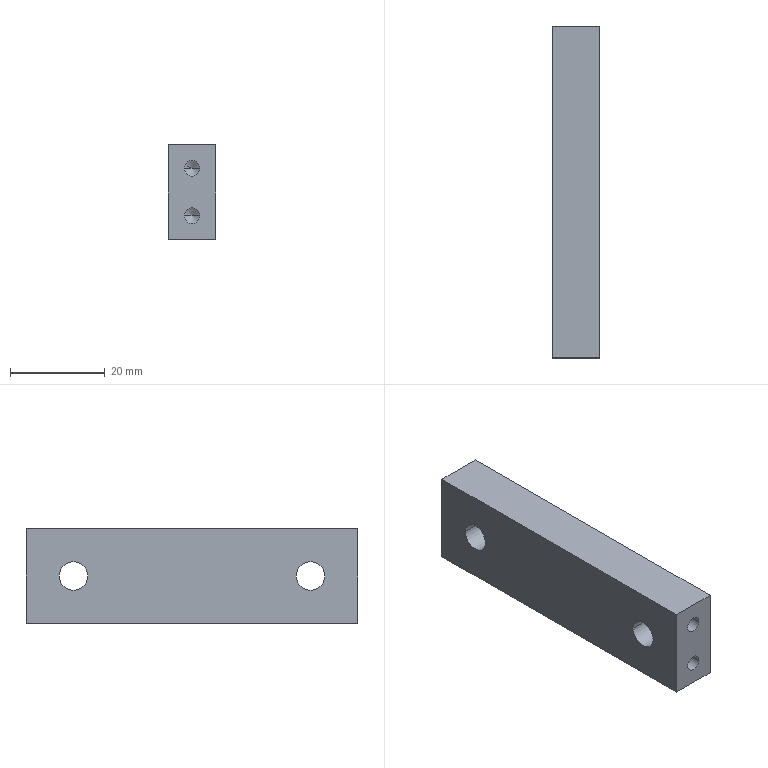Component | SolidWorks | EpoxyBoardSupportBlock-1 | 1 solid | 26 faces | box 10 x 70 x 20 mm | volume 13010 mm3 | cylinder 12 | cone 8 | plane 6 | commonest cylinder face diameters 3.3 x8 6 x4
build123d program:
from build123d import *

# Parameters (mm, degrees)
SKETCH1_W             = 70
SKETCH1_H             = 20
BOSS_EXTRUDE1_DEPTH   = 5
M6_TAPPED_HOLE1_D     = 6
M4_TAPPED_HOLE1_D     = 3.3
M4_TAPPED_HOLE1_DEPTH = 12.1
M4_TAPPED_HOLE1_TIP   = 0.9526
M4_TAPPED_HOLE2_D     = 3.3
M4_TAPPED_HOLE2_DEPTH = 12.1
M4_TAPPED_HOLE2_TIP   = 0.9526


with BuildPart() as part:
    # Sketch1 → Boss-Extrude1 (new, symmetric)
    with BuildSketch(Plane.XY):
        with Locations((35, 10)):
            Rectangle(SKETCH1_W, SKETCH1_H)
    extrude(amount=BOSS_EXTRUDE1_DEPTH, both=True)

    # M6 Tapped Hole1 (through all)
    with Locations(Plane(origin=(10, 10, 5), x_dir=(1, 0, 0), z_dir=(0, 0, 1))):
        with Locations((0, 0), (50, 0)):
            Hole(M6_TAPPED_HOLE1_D / 2)

    # M4 Tapped Hole1
    with Locations(Plane(origin=(0, 15, 0), x_dir=(0, 0, -1), z_dir=(-1, 0, 0))):
        with Locations((0, 0), (0, 10)):
            Hole(M4_TAPPED_HOLE1_D / 2, depth=M4_TAPPED_HOLE1_DEPTH)
            with Locations((0, 0, -(M4_TAPPED_HOLE1_DEPTH + M4_TAPPED_HOLE1_TIP / 2))):  # 120° drill point
                Cone(0, M4_TAPPED_HOLE1_D / 2, M4_TAPPED_HOLE1_TIP, mode=Mode.SUBTRACT)

    # M4 Tapped Hole2
    with Locations(Plane(origin=(70, 15, 0), x_dir=(0, 0, 1), z_dir=(1, 0, 0))):
        with Locations((0, 0), (0, 10)):
            Hole(M4_TAPPED_HOLE2_D / 2, depth=M4_TAPPED_HOLE2_DEPTH)
            with Locations((0, 0, -(M4_TAPPED_HOLE2_DEPTH + M4_TAPPED_HOLE2_TIP / 2))):  # 120° drill point
                Cone(0, M4_TAPPED_HOLE2_D / 2, M4_TAPPED_HOLE2_TIP, mode=Mode.SUBTRACT)


solid = part.part

# Placed as in the assembly
solid = solid.moved(Location((-28.341, 72.185, -51.775), (90, -90, 0)))
STEP:
#1=COLOUR_RGB('',0.7922,0.8196,0.9333);
#2=FILL_AREA_STYLE_COLOUR('',#1);
#3=FILL_AREA_STYLE('',(#2));
#4=SURFACE_STYLE_FILL_AREA(#3);
#5=SURFACE_SIDE_STYLE('',(#4));
#6=SURFACE_STYLE_USAGE(.BOTH.,#5);
#7=PRESENTATION_STYLE_ASSIGNMENT((#6));
#8=CARTESIAN_POINT('',(-1.051,0.5624,-1.842));
#9=VERTEX_POINT('',#8);
#10=CARTESIAN_POINT('',(-1.181,0.5624,-1.842));
#11=VERTEX_POINT('',#10);
#12=CARTESIAN_POINT('',(-1.116,0.5624,-1.842));
#13=DIRECTION('',(0.,-1.,0.));
#14=DIRECTION('',(-1.,0.,0.));
#15=AXIS2_PLACEMENT_3D('',#12,#13,#14);
#16=CIRCLE('',#15,0.06496);
#17=EDGE_CURVE('',#9,#11,#16,.T.);
#18=ORIENTED_EDGE('',*,*,#17,.F.);
#19=CARTESIAN_POINT('',(-1.051,0.08603,-1.842));
#20=VERTEX_POINT('',#19);
#21=CARTESIAN_POINT('',(-1.051,0.08603,-1.842));
#22=DIRECTION('',(0.,-1.,0.));
#23=VECTOR('',#22,39.37);
#24=LINE('',#21,#23);
#25=EDGE_CURVE('',#9,#20,#24,.T.);
#26=ORIENTED_EDGE('',*,*,#25,.T.);
#27=CARTESIAN_POINT('',(-1.181,0.08603,-1.842));
#28=VERTEX_POINT('',#27);
#29=CARTESIAN_POINT('',(-1.116,0.08603,-1.842));
#30=DIRECTION('',(0.,-1.,0.));
#31=DIRECTION('',(-1.,0.,0.));
#32=AXIS2_PLACEMENT_3D('',#29,#30,#31);
#33=CIRCLE('',#32,0.06496);
#34=EDGE_CURVE('',#20,#28,#33,.T.);
#35=ORIENTED_EDGE('',*,*,#34,.T.);
#36=CARTESIAN_POINT('',(-1.181,0.08603,-1.842));
#37=DIRECTION('',(0.,-1.,0.));
#38=VECTOR('',#37,39.37);
#39=LINE('',#36,#38);
#40=EDGE_CURVE('',#11,#28,#39,.T.);
#41=ORIENTED_EDGE('',*,*,#40,.F.);
#42=EDGE_LOOP('',(#18,#26,#35,#41));
#43=FACE_OUTER_BOUND('',#42,.T.);
#44=CARTESIAN_POINT('',(-1.116,0.08603,-1.842));
#45=DIRECTION('',(0.,-1.,0.));
#46=DIRECTION('',(-1.,0.,0.));
#47=AXIS2_PLACEMENT_3D('',#44,#45,#46);
#48=CYLINDRICAL_SURFACE('',#47,0.06496);
#49=ADVANCED_FACE('',(#43),#48,.F.);
#50=CARTESIAN_POINT('',(-1.116,0.5999,-1.842));
#51=VERTEX_POINT('',#50);
#52=CARTESIAN_POINT('',(-1.181,0.5624,-1.842));
#53=DIRECTION('',(-0.866,-0.5,0.));
#54=VECTOR('',#53,39.37);
#55=LINE('',#52,#54);
#56=EDGE_CURVE('',#51,#11,#55,.T.);
#57=ORIENTED_EDGE('',*,*,#56,.F.);
#58=CARTESIAN_POINT('',(-1.051,0.5624,-1.842));
#59=DIRECTION('',(0.866,-0.5,0.));
#60=VECTOR('',#59,39.37);
#61=LINE('',#58,#60);
#62=EDGE_CURVE('',#51,#9,#61,.T.);
#63=ORIENTED_EDGE('',*,*,#62,.T.);
#64=ORIENTED_EDGE('',*,*,#17,.T.);
#65=EDGE_LOOP('',(#57,#63,#64));
#66=FACE_OUTER_BOUND('',#65,.T.);
#67=CARTESIAN_POINT('',(-1.116,0.5624,-1.842));
#68=DIRECTION('',(0.,-1.,0.));
#69=DIRECTION('',(-1.,0.,0.));
#70=AXIS2_PLACEMENT_3D('',#67,#68,#69);
#71=CONICAL_SURFACE('',#70,0.06496,1.047);
#72=ADVANCED_FACE('',(#66),#71,.F.);
#73=CARTESIAN_POINT('',(-1.051,0.5624,-1.448));
#74=VERTEX_POINT('',#73);
#75=CARTESIAN_POINT('',(-1.181,0.5624,-1.448));
#76=VERTEX_POINT('',#75);
#77=CARTESIAN_POINT('',(-1.116,0.5624,-1.448));
#78=DIRECTION('',(0.,-1.,0.));
#79=DIRECTION('',(-1.,0.,0.));
#80=AXIS2_PLACEMENT_3D('',#77,#78,#79);
#81=CIRCLE('',#80,0.06496);
#82=EDGE_CURVE('',#74,#76,#81,.T.);
#83=ORIENTED_EDGE('',*,*,#82,.F.);
#84=CARTESIAN_POINT('',(-1.051,0.08603,-1.448));
#85=VERTEX_POINT('',#84);
#86=CARTESIAN_POINT('',(-1.051,0.08603,-1.448));
#87=DIRECTION('',(0.,-1.,0.));
#88=VECTOR('',#87,39.37);
#89=LINE('',#86,#88);
#90=EDGE_CURVE('',#74,#85,#89,.T.);
#91=ORIENTED_EDGE('',*,*,#90,.T.);
#92=CARTESIAN_POINT('',(-1.181,0.08603,-1.448));
#93=VERTEX_POINT('',#92);
#94=CARTESIAN_POINT('',(-1.116,0.08603,-1.448));
#95=DIRECTION('',(0.,-1.,0.));
#96=DIRECTION('',(-1.,0.,0.));
#97=AXIS2_PLACEMENT_3D('',#94,#95,#96);
#98=CIRCLE('',#97,0.06496);
#99=EDGE_CURVE('',#85,#93,#98,.T.);
#100=ORIENTED_EDGE('',*,*,#99,.T.);
#101=CARTESIAN_POINT('',(-1.181,0.08603,-1.448));
#102=DIRECTION('',(0.,-1.,0.));
#103=VECTOR('',#102,39.37);
#104=LINE('',#101,#103);
#105=EDGE_CURVE('',#76,#93,#104,.T.);
#106=ORIENTED_EDGE('',*,*,#105,.F.);
#107=EDGE_LOOP('',(#83,#91,#100,#106));
#108=FACE_OUTER_BOUND('',#107,.T.);
#109=CARTESIAN_POINT('',(-1.116,0.08603,-1.448));
#110=DIRECTION('',(0.,-1.,0.));
#111=DIRECTION('',(-1.,0.,0.));
#112=AXIS2_PLACEMENT_3D('',#109,#110,#111);
#113=CYLINDRICAL_SURFACE('',#112,0.06496);
#114=ADVANCED_FACE('',(#108),#113,.F.);
#115=CARTESIAN_POINT('',(-1.116,0.5999,-1.448));
#116=VERTEX_POINT('',#115);
#117=CARTESIAN_POINT('',(-1.181,0.5624,-1.448));
#118=DIRECTION('',(-0.866,-0.5,0.));
#119=VECTOR('',#118,39.37);
#120=LINE('',#117,#119);
#121=EDGE_CURVE('',#116,#76,#120,.T.);
#122=ORIENTED_EDGE('',*,*,#121,.F.);
#123=CARTESIAN_POINT('',(-1.051,0.5624,-1.448));
#124=DIRECTION('',(0.866,-0.5,0.));
#125=VECTOR('',#124,39.37);
#126=LINE('',#123,#125);
#127=EDGE_CURVE('',#116,#74,#126,.T.);
#128=ORIENTED_EDGE('',*,*,#127,.T.);
#129=ORIENTED_EDGE('',*,*,#82,.T.);
#130=EDGE_LOOP('',(#122,#128,#129));
#131=FACE_OUTER_BOUND('',#130,.T.);
#132=CARTESIAN_POINT('',(-1.116,0.5624,-1.448));
#133=DIRECTION('',(0.,-1.,0.));
#134=DIRECTION('',(-1.,0.,0.));
#135=AXIS2_PLACEMENT_3D('',#132,#133,#134);
#136=CONICAL_SURFACE('',#135,0.06496,1.047);
#137=ADVANCED_FACE('',(#131),#136,.F.);
#138=CARTESIAN_POINT('',(-1.181,2.366,-1.842));
#139=VERTEX_POINT('',#138);
#140=CARTESIAN_POINT('',(-1.051,2.366,-1.842));
#141=VERTEX_POINT('',#140);
#142=CARTESIAN_POINT('',(-1.116,2.366,-1.842));
#143=DIRECTION('',(-0.,1.,-0.));
#144=DIRECTION('',(1.,0.,0.));
#145=AXIS2_PLACEMENT_3D('',#142,#143,#144);
#146=CIRCLE('',#145,0.06496);
#147=EDGE_CURVE('',#139,#141,#146,.T.);
#148=ORIENTED_EDGE('',*,*,#147,.F.);
#149=CARTESIAN_POINT('',(-1.181,2.842,-1.842));
#150=VERTEX_POINT('',#149);
#151=CARTESIAN_POINT('',(-1.181,2.842,-1.842));
#152=DIRECTION('',(-0.,1.,-0.));
#153=VECTOR('',#152,39.37);
#154=LINE('',#151,#153);
#155=EDGE_CURVE('',#139,#150,#154,.T.);
#156=ORIENTED_EDGE('',*,*,#155,.T.);
#157=CARTESIAN_POINT('',(-1.051,2.842,-1.842));
#158=VERTEX_POINT('',#157);
#159=CARTESIAN_POINT('',(-1.116,2.842,-1.842));
#160=DIRECTION('',(-0.,1.,-0.));
#161=DIRECTION('',(1.,0.,0.));
#162=AXIS2_PLACEMENT_3D('',#159,#160,#161);
#163=CIRCLE('',#162,0.06496);
#164=EDGE_CURVE('',#150,#158,#163,.T.);
#165=ORIENTED_EDGE('',*,*,#164,.T.);
#166=CARTESIAN_POINT('',(-1.051,2.842,-1.842));
#167=DIRECTION('',(-0.,1.,-0.));
#168=VECTOR('',#167,39.37);
#169=LINE('',#166,#168);
#170=EDGE_CURVE('',#141,#158,#169,.T.);
#171=ORIENTED_EDGE('',*,*,#170,.F.);
#172=EDGE_LOOP('',(#148,#156,#165,#171));
#173=FACE_OUTER_BOUND('',#172,.T.);
#174=CARTESIAN_POINT('',(-1.116,2.842,-1.842));
#175=DIRECTION('',(-0.,1.,-0.));
#176=DIRECTION('',(1.,0.,0.));
#177=AXIS2_PLACEMENT_3D('',#174,#175,#176);
#178=CYLINDRICAL_SURFACE('',#177,0.06496);
#179=ADVANCED_FACE('',(#173),#178,.F.);
#180=CARTESIAN_POINT('',(-1.116,2.328,-1.842));
#181=VERTEX_POINT('',#180);
#182=CARTESIAN_POINT('',(-1.051,2.366,-1.842));
#183=DIRECTION('',(0.866,0.5,-0.));
#184=VECTOR('',#183,39.37);
#185=LINE('',#182,#184);
#186=EDGE_CURVE('',#181,#141,#185,.T.);
#187=ORIENTED_EDGE('',*,*,#186,.F.);
#188=CARTESIAN_POINT('',(-1.181,2.366,-1.842));
#189=DIRECTION('',(-0.866,0.5,-0.));
#190=VECTOR('',#189,39.37);
#191=LINE('',#188,#190);
#192=EDGE_CURVE('',#181,#139,#191,.T.);
#193=ORIENTED_EDGE('',*,*,#192,.T.);
#194=ORIENTED_EDGE('',*,*,#147,.T.);
#195=EDGE_LOOP('',(#187,#193,#194));
#196=FACE_OUTER_BOUND('',#195,.T.);
#197=CARTESIAN_POINT('',(-1.116,2.366,-1.842));
#198=DIRECTION('',(-0.,1.,-0.));
#199=DIRECTION('',(1.,0.,0.));
#200=AXIS2_PLACEMENT_3D('',#197,#198,#199);
#201=CONICAL_SURFACE('',#200,0.06496,1.047);
#202=ADVANCED_FACE('',(#196),#201,.F.);
#203=CARTESIAN_POINT('',(-1.181,2.366,-1.448));
#204=VERTEX_POINT('',#203);
#205=CARTESIAN_POINT('',(-1.051,2.366,-1.448));
#206=VERTEX_POINT('',#205);
#207=CARTESIAN_POINT('',(-1.116,2.366,-1.448));
#208=DIRECTION('',(-0.,1.,-0.));
#209=DIRECTION('',(1.,0.,0.));
#210=AXIS2_PLACEMENT_3D('',#207,#208,#209);
#211=CIRCLE('',#210,0.06496);
#212=EDGE_CURVE('',#204,#206,#211,.T.);
#213=ORIENTED_EDGE('',*,*,#212,.F.);
#214=CARTESIAN_POINT('',(-1.181,2.842,-1.448));
#215=VERTEX_POINT('',#214);
#216=CARTESIAN_POINT('',(-1.181,2.842,-1.448));
#217=DIRECTION('',(-0.,1.,-0.));
#218=VECTOR('',#217,39.37);
#219=LINE('',#216,#218);
#220=EDGE_CURVE('',#204,#215,#219,.T.);
#221=ORIENTED_EDGE('',*,*,#220,.T.);
#222=CARTESIAN_POINT('',(-1.051,2.842,-1.448));
#223=VERTEX_POINT('',#222);
#224=CARTESIAN_POINT('',(-1.116,2.842,-1.448));
#225=DIRECTION('',(-0.,1.,-0.));
#226=DIRECTION('',(1.,0.,0.));
#227=AXIS2_PLACEMENT_3D('',#224,#225,#226);
#228=CIRCLE('',#227,0.06496);
#229=EDGE_CURVE('',#215,#223,#228,.T.);
#230=ORIENTED_EDGE('',*,*,#229,.T.);
#231=CARTESIAN_POINT('',(-1.051,2.842,-1.448));
#232=DIRECTION('',(-0.,1.,-0.));
#233=VECTOR('',#232,39.37);
#234=LINE('',#231,#233);
#235=EDGE_CURVE('',#206,#223,#234,.T.);
#236=ORIENTED_EDGE('',*,*,#235,.F.);
#237=EDGE_LOOP('',(#213,#221,#230,#236));
#238=FACE_OUTER_BOUND('',#237,.T.);
#239=CARTESIAN_POINT('',(-1.116,2.842,-1.448));
#240=DIRECTION('',(-0.,1.,-0.));
#241=DIRECTION('',(1.,0.,0.));
#242=AXIS2_PLACEMENT_3D('',#239,#240,#241);
#243=CYLINDRICAL_SURFACE('',#242,0.06496);
#244=ADVANCED_FACE('',(#238),#243,.F.);
#245=CARTESIAN_POINT('',(-1.116,2.328,-1.448));
#246=VERTEX_POINT('',#245);
#247=CARTESIAN_POINT('',(-1.051,2.366,-1.448));
#248=DIRECTION('',(0.866,0.5,-0.));
#249=VECTOR('',#248,39.37);
#250=LINE('',#247,#249);
#251=EDGE_CURVE('',#246,#206,#250,.T.);
#252=ORIENTED_EDGE('',*,*,#251,.F.);
#253=CARTESIAN_POINT('',(-1.181,2.366,-1.448));
#254=DIRECTION('',(-0.866,0.5,-0.));
#255=VECTOR('',#254,39.37);
#256=LINE('',#253,#255);
#257=EDGE_CURVE('',#246,#204,#256,.T.);
#258=ORIENTED_EDGE('',*,*,#257,.T.);
#259=ORIENTED_EDGE('',*,*,#212,.T.);
#260=EDGE_LOOP('',(#252,#258,#259));
#261=FACE_OUTER_BOUND('',#260,.T.);
#262=CARTESIAN_POINT('',(-1.116,2.366,-1.448));
#263=DIRECTION('',(-0.,1.,-0.));
#264=DIRECTION('',(1.,0.,0.));
#265=AXIS2_PLACEMENT_3D('',#262,#263,#264);
#266=CONICAL_SURFACE('',#265,0.06496,1.047);
#267=ADVANCED_FACE('',(#261),#266,.F.);
#268=CARTESIAN_POINT('',(-1.313,2.566,-1.645));
#269=VERTEX_POINT('',#268);
#270=CARTESIAN_POINT('',(-1.313,2.33,-1.645));
#271=VERTEX_POINT('',#270);
#272=CARTESIAN_POINT('',(-1.313,2.448,-1.645));
#273=DIRECTION('',(1.,0.,-0.));
#274=DIRECTION('',(0.,-1.,0.));
#275=AXIS2_PLACEMENT_3D('',#272,#273,#274);
#276=CIRCLE('',#275,0.1181);
#277=EDGE_CURVE('',#269,#271,#276,.T.);
#278=ORIENTED_EDGE('',*,*,#277,.F.);
#279=CARTESIAN_POINT('',(-0.919,2.566,-1.645));
#280=VERTEX_POINT('',#279);
#281=CARTESIAN_POINT('',(-0.919,2.566,-1.645));
#282=DIRECTION('',(1.,0.,-0.));
#283=VECTOR('',#282,39.37);
#284=LINE('',#281,#283);
#285=EDGE_CURVE('',#269,#280,#284,.T.);
#286=ORIENTED_EDGE('',*,*,#285,.T.);
#287=CARTESIAN_POINT('',(-0.919,2.33,-1.645));
#288=VERTEX_POINT('',#287);
#289=CARTESIAN_POINT('',(-0.919,2.448,-1.645));
#290=DIRECTION('',(1.,0.,-0.));
#291=DIRECTION('',(0.,-1.,0.));
#292=AXIS2_PLACEMENT_3D('',#289,#290,#291);
#293=CIRCLE('',#292,0.1181);
#294=EDGE_CURVE('',#280,#288,#293,.T.);
#295=ORIENTED_EDGE('',*,*,#294,.T.);
#296=CARTESIAN_POINT('',(-0.919,2.33,-1.645));
#297=DIRECTION('',(1.,0.,-0.));
#298=VECTOR('',#297,39.37);
#299=LINE('',#296,#298);
#300=EDGE_CURVE('',#271,#288,#299,.T.);
#301=ORIENTED_EDGE('',*,*,#300,.F.);
#302=EDGE_LOOP('',(#278,#286,#295,#301));
#303=FACE_OUTER_BOUND('',#302,.T.);
#304=CARTESIAN_POINT('',(-0.919,2.448,-1.645));
#305=DIRECTION('',(1.,0.,-0.));
#306=DIRECTION('',(0.,-1.,0.));
#307=AXIS2_PLACEMENT_3D('',#304,#305,#306);
#308=CYLINDRICAL_SURFACE('',#307,0.1181);
#309=ADVANCED_FACE('',(#303),#308,.F.);
#310=CARTESIAN_POINT('',(-1.313,0.5978,-1.645));
#311=VERTEX_POINT('',#310);
#312=CARTESIAN_POINT('',(-1.313,0.3616,-1.645));
#313=VERTEX_POINT('',#312);
#314=CARTESIAN_POINT('',(-1.313,0.4797,-1.645));
#315=DIRECTION('',(1.,0.,-0.));
#316=DIRECTION('',(0.,-1.,0.));
#317=AXIS2_PLACEMENT_3D('',#314,#315,#316);
#318=CIRCLE('',#317,0.1181);
#319=EDGE_CURVE('',#311,#313,#318,.T.);
#320=ORIENTED_EDGE('',*,*,#319,.F.);
#321=CARTESIAN_POINT('',(-0.919,0.5978,-1.645));
#322=VERTEX_POINT('',#321);
#323=CARTESIAN_POINT('',(-0.919,0.5978,-1.645));
#324=DIRECTION('',(1.,0.,-0.));
#325=VECTOR('',#324,39.37);
#326=LINE('',#323,#325);
#327=EDGE_CURVE('',#311,#322,#326,.T.);
#328=ORIENTED_EDGE('',*,*,#327,.T.);
#329=CARTESIAN_POINT('',(-0.919,0.3616,-1.645));
#330=VERTEX_POINT('',#329);
#331=CARTESIAN_POINT('',(-0.919,0.4797,-1.645));
#332=DIRECTION('',(1.,0.,-0.));
#333=DIRECTION('',(0.,-1.,0.));
#334=AXIS2_PLACEMENT_3D('',#331,#332,#333);
#335=CIRCLE('',#334,0.1181);
#336=EDGE_CURVE('',#322,#330,#335,.T.);
#337=ORIENTED_EDGE('',*,*,#336,.T.);
#338=CARTESIAN_POINT('',(-0.919,0.3616,-1.645));
#339=DIRECTION('',(1.,0.,-0.));
#340=VECTOR('',#339,39.37);
#341=LINE('',#338,#340);
#342=EDGE_CURVE('',#313,#330,#341,.T.);
#343=ORIENTED_EDGE('',*,*,#342,.F.);
#344=EDGE_LOOP('',(#320,#328,#337,#343));
#345=FACE_OUTER_BOUND('',#344,.T.);
#346=CARTESIAN_POINT('',(-0.919,0.4797,-1.645));
#347=DIRECTION('',(1.,0.,-0.));
#348=DIRECTION('',(0.,-1.,0.));
#349=AXIS2_PLACEMENT_3D('',#346,#347,#348);
#350=CYLINDRICAL_SURFACE('',#349,0.1181);
#351=ADVANCED_FACE('',(#345),#350,.F.);
#352=CARTESIAN_POINT('',(-1.116,2.842,-1.842));
#353=DIRECTION('',(-0.,1.,-0.));
#354=DIRECTION('',(1.,0.,0.));
#355=AXIS2_PLACEMENT_3D('',#352,#353,#354);
#356=CIRCLE('',#355,0.06496);
#357=EDGE_CURVE('',#158,#150,#356,.T.);
#358=ORIENTED_EDGE('',*,*,#357,.F.);
#359=ORIENTED_EDGE('',*,*,#164,.F.);
#360=EDGE_LOOP('',(#358,#359));
#361=FACE_BOUND('',#360,.T.);
#362=CARTESIAN_POINT('',(-1.116,2.842,-1.448));
#363=DIRECTION('',(-0.,1.,-0.));
#364=DIRECTION('',(1.,0.,0.));
#365=AXIS2_PLACEMENT_3D('',#362,#363,#364);
#366=CIRCLE('',#365,0.06496);
#367=EDGE_CURVE('',#223,#215,#366,.T.);
#368=ORIENTED_EDGE('',*,*,#367,.F.);
#369=ORIENTED_EDGE('',*,*,#229,.F.);
#370=EDGE_LOOP('',(#368,#369));
#371=FACE_BOUND('',#370,.T.);
#372=CARTESIAN_POINT('',(-1.313,2.842,-2.038));
#373=VERTEX_POINT('',#372);
#374=CARTESIAN_POINT('',(-1.313,2.842,-1.251));
#375=VERTEX_POINT('',#374);
#376=CARTESIAN_POINT('',(-1.313,2.842,-1.251));
#377=DIRECTION('',(0.,0.,1.));
#378=VECTOR('',#377,39.37);
#379=LINE('',#376,#378);
#380=EDGE_CURVE('',#373,#375,#379,.T.);
#381=ORIENTED_EDGE('',*,*,#380,.T.);
#382=CARTESIAN_POINT('',(-0.919,2.842,-1.251));
#383=VERTEX_POINT('',#382);
#384=CARTESIAN_POINT('',(-0.919,2.842,-1.251));
#385=DIRECTION('',(-1.,-0.,0.));
#386=VECTOR('',#385,39.37);
#387=LINE('',#384,#386);
#388=EDGE_CURVE('',#383,#375,#387,.T.);
#389=ORIENTED_EDGE('',*,*,#388,.F.);
#390=CARTESIAN_POINT('',(-0.919,2.842,-2.038));
#391=VERTEX_POINT('',#390);
#392=CARTESIAN_POINT('',(-0.919,2.842,-1.251));
#393=DIRECTION('',(0.,0.,1.));
#394=VECTOR('',#393,39.37);
#395=LINE('',#392,#394);
#396=EDGE_CURVE('',#391,#383,#395,.T.);
#397=ORIENTED_EDGE('',*,*,#396,.F.);
#398=CARTESIAN_POINT('',(-0.919,2.842,-2.038));
#399=DIRECTION('',(-1.,-0.,0.));
#400=VECTOR('',#399,39.37);
#401=LINE('',#398,#400);
#402=EDGE_CURVE('',#391,#373,#401,.T.);
#403=ORIENTED_EDGE('',*,*,#402,.T.);
#404=EDGE_LOOP('',(#381,#389,#397,#403));
#405=FACE_OUTER_BOUND('',#404,.T.);
#406=CARTESIAN_POINT('',(-0.919,2.842,-1.251));
#407=DIRECTION('',(0.,-1.,0.));
#408=DIRECTION('',(-1.,-0.,0.));
#409=AXIS2_PLACEMENT_3D('',#406,#407,#408);
#410=PLANE('',#409);
#411=ADVANCED_FACE('',(#361,#371,#405),#410,.F.);
#412=CARTESIAN_POINT('',(-1.313,0.08603,-1.251));
#413=VERTEX_POINT('',#412);
#414=CARTESIAN_POINT('',(-1.313,2.842,-1.251));
#415=DIRECTION('',(0.,-1.,0.));
#416=VECTOR('',#415,39.37);
#417=LINE('',#414,#416);
#418=EDGE_CURVE('',#375,#413,#417,.T.);
#419=ORIENTED_EDGE('',*,*,#418,.T.);
#420=CARTESIAN_POINT('',(-0.919,0.08603,-1.251));
#421=VERTEX_POINT('',#420);
#422=CARTESIAN_POINT('',(-0.919,0.08603,-1.251));
#423=DIRECTION('',(-1.,-0.,0.));
#424=VECTOR('',#423,39.37);
#425=LINE('',#422,#424);
#426=EDGE_CURVE('',#421,#413,#425,.T.);
#427=ORIENTED_EDGE('',*,*,#426,.F.);
#428=CARTESIAN_POINT('',(-0.919,2.842,-1.251));
#429=DIRECTION('',(0.,-1.,0.));
#430=VECTOR('',#429,39.37);
#431=LINE('',#428,#430);
#432=EDGE_CURVE('',#383,#421,#431,.T.);
#433=ORIENTED_EDGE('',*,*,#432,.F.);
#434=ORIENTED_EDGE('',*,*,#388,.T.);
#435=EDGE_LOOP('',(#419,#427,#433,#434));
#436=FACE_OUTER_BOUND('',#435,.T.);
#437=CARTESIAN_POINT('',(-0.919,2.842,-1.251));
#438=DIRECTION('',(-0.,-0.,-1.));
#439=DIRECTION('',(1.,0.,-0.));
#440=AXIS2_PLACEMENT_3D('',#437,#438,#439);
#441=PLANE('',#440);
#442=ADVANCED_FACE('',(#436),#441,.F.);
#443=CARTESIAN_POINT('',(-1.116,0.08603,-1.842));
#444=DIRECTION('',(0.,-1.,0.));
#445=DIRECTION('',(-1.,0.,0.));
#446=AXIS2_PLACEMENT_3D('',#443,#444,#445);
#447=CIRCLE('',#446,0.06496);
#448=EDGE_CURVE('',#28,#20,#447,.T.);
#449=ORIENTED_EDGE('',*,*,#448,.F.);
#450=ORIENTED_EDGE('',*,*,#34,.F.);
#451=EDGE_LOOP('',(#449,#450));
#452=FACE_BOUND('',#451,.T.);
#453=CARTESIAN_POINT('',(-1.116,0.08603,-1.448));
#454=DIRECTION('',(0.,-1.,0.));
#455=DIRECTION('',(-1.,0.,0.));
#456=AXIS2_PLACEMENT_3D('',#453,#454,#455);
#457=CIRCLE('',#456,0.06496);
#458=EDGE_CURVE('',#93,#85,#457,.T.);
#459=ORIENTED_EDGE('',*,*,#458,.F.);
#460=ORIENTED_EDGE('',*,*,#99,.F.);
#461=EDGE_LOOP('',(#459,#460));
#462=FACE_BOUND('',#461,.T.);
#463=CARTESIAN_POINT('',(-1.313,0.08603,-2.038));
#464=VERTEX_POINT('',#463);
#465=CARTESIAN_POINT('',(-1.313,0.08603,-1.251));
#466=DIRECTION('',(-0.,-0.,-1.));
#467=VECTOR('',#466,39.37);
#468=LINE('',#465,#467);
#469=EDGE_CURVE('',#413,#464,#468,.T.);
#470=ORIENTED_EDGE('',*,*,#469,.T.);
#471=CARTESIAN_POINT('',(-0.919,0.08603,-2.038));
#472=VERTEX_POINT('',#471);
#473=CARTESIAN_POINT('',(-0.919,0.08603,-2.038));
#474=DIRECTION('',(-1.,-0.,0.));
#475=VECTOR('',#474,39.37);
#476=LINE('',#473,#475);
#477=EDGE_CURVE('',#472,#464,#476,.T.);
#478=ORIENTED_EDGE('',*,*,#477,.F.);
#479=CARTESIAN_POINT('',(-0.919,0.08603,-1.251));
#480=DIRECTION('',(-0.,-0.,-1.));
#481=VECTOR('',#480,39.37);
#482=LINE('',#479,#481);
#483=EDGE_CURVE('',#421,#472,#482,.T.);
#484=ORIENTED_EDGE('',*,*,#483,.F.);
#485=ORIENTED_EDGE('',*,*,#426,.T.);
#486=EDGE_LOOP('',(#470,#478,#484,#485));
#487=FACE_OUTER_BOUND('',#486,.T.);
#488=CARTESIAN_POINT('',(-0.919,0.08603,-1.251));
#489=DIRECTION('',(-0.,1.,-0.));
#490=DIRECTION('',(1.,0.,-0.));
#491=AXIS2_PLACEMENT_3D('',#488,#489,#490);
#492=PLANE('',#491);
#493=ADVANCED_FACE('',(#452,#462,#487),#492,.F.);
#494=CARTESIAN_POINT('',(-1.313,2.842,-2.038));
#495=DIRECTION('',(-0.,1.,-0.));
#496=VECTOR('',#495,39.37);
#497=LINE('',#494,#496);
#498=EDGE_CURVE('',#464,#373,#497,.T.);
#499=ORIENTED_EDGE('',*,*,#498,.T.);
#500=ORIENTED_EDGE('',*,*,#402,.F.);
#501=CARTESIAN_POINT('',(-0.919,2.842,-2.038));
#502=DIRECTION('',(-0.,1.,-0.));
#503=VECTOR('',#502,39.37);
#504=LINE('',#501,#503);
#505=EDGE_CURVE('',#472,#391,#504,.T.);
#506=ORIENTED_EDGE('',*,*,#505,.F.);
#507=ORIENTED_EDGE('',*,*,#477,.T.);
#508=EDGE_LOOP('',(#499,#500,#506,#507));
#509=FACE_OUTER_BOUND('',#508,.T.);
#510=CARTESIAN_POINT('',(-0.919,2.842,-2.038));
#511=DIRECTION('',(0.,0.,1.));
#512=DIRECTION('',(-1.,-0.,0.));
#513=AXIS2_PLACEMENT_3D('',#510,#511,#512);
#514=PLANE('',#513);
#515=ADVANCED_FACE('',(#509),#514,.F.);
#516=CARTESIAN_POINT('',(-0.919,2.448,-1.645));
#517=DIRECTION('',(1.,0.,-0.));
#518=DIRECTION('',(0.,-1.,0.));
#519=AXIS2_PLACEMENT_3D('',#516,#517,#518);
#520=CIRCLE('',#519,0.1181);
#521=EDGE_CURVE('',#288,#280,#520,.T.);
#522=ORIENTED_EDGE('',*,*,#521,.F.);
#523=ORIENTED_EDGE('',*,*,#294,.F.);
#524=EDGE_LOOP('',(#522,#523));
#525=FACE_BOUND('',#524,.T.);
#526=CARTESIAN_POINT('',(-0.919,0.4797,-1.645));
#527=DIRECTION('',(1.,0.,-0.));
#528=DIRECTION('',(0.,-1.,0.));
#529=AXIS2_PLACEMENT_3D('',#526,#527,#528);
#530=CIRCLE('',#529,0.1181);
#531=EDGE_CURVE('',#330,#322,#530,.T.);
#532=ORIENTED_EDGE('',*,*,#531,.F.);
#533=ORIENTED_EDGE('',*,*,#336,.F.);
#534=EDGE_LOOP('',(#532,#533));
#535=FACE_BOUND('',#534,.T.);
#536=ORIENTED_EDGE('',*,*,#396,.T.);
#537=ORIENTED_EDGE('',*,*,#432,.T.);
#538=ORIENTED_EDGE('',*,*,#483,.T.);
#539=ORIENTED_EDGE('',*,*,#505,.T.);
#540=EDGE_LOOP('',(#536,#537,#538,#539));
#541=FACE_OUTER_BOUND('',#540,.T.);
#542=CARTESIAN_POINT('',(-0.919,2.842,-1.251));
#543=DIRECTION('',(-1.,-0.,0.));
#544=DIRECTION('',(-0.,1.,-0.));
#545=AXIS2_PLACEMENT_3D('',#542,#543,#544);
#546=PLANE('',#545);
#547=ADVANCED_FACE('',(#525,#535,#541),#546,.F.);
#548=CARTESIAN_POINT('',(-1.313,2.448,-1.645));
#549=DIRECTION('',(1.,0.,-0.));
#550=DIRECTION('',(0.,-1.,0.));
#551=AXIS2_PLACEMENT_3D('',#548,#549,#550);
#552=CIRCLE('',#551,0.1181);
#553=EDGE_CURVE('',#271,#269,#552,.T.);
#554=ORIENTED_EDGE('',*,*,#553,.T.);
#555=ORIENTED_EDGE('',*,*,#277,.T.);
#556=EDGE_LOOP('',(#554,#555));
#557=FACE_BOUND('',#556,.T.);
#558=CARTESIAN_POINT('',(-1.313,0.4797,-1.645));
#559=DIRECTION('',(1.,0.,-0.));
#560=DIRECTION('',(0.,-1.,0.));
#561=AXIS2_PLACEMENT_3D('',#558,#559,#560);
#562=CIRCLE('',#561,0.1181);
#563=EDGE_CURVE('',#313,#311,#562,.T.);
#564=ORIENTED_EDGE('',*,*,#563,.T.);
#565=ORIENTED_EDGE('',*,*,#319,.T.);
#566=EDGE_LOOP('',(#564,#565));
#567=FACE_BOUND('',#566,.T.);
#568=ORIENTED_EDGE('',*,*,#380,.F.);
#569=ORIENTED_EDGE('',*,*,#498,.F.);
#570=ORIENTED_EDGE('',*,*,#469,.F.);
#571=ORIENTED_EDGE('',*,*,#418,.F.);
#572=EDGE_LOOP('',(#568,#569,#570,#571));
#573=FACE_OUTER_BOUND('',#572,.T.);
#574=CARTESIAN_POINT('',(-1.313,2.842,-1.251));
#575=DIRECTION('',(-1.,-0.,0.));
#576=DIRECTION('',(-0.,1.,-0.));
#577=AXIS2_PLACEMENT_3D('',#574,#575,#576);
#578=PLANE('',#577);
#579=ADVANCED_FACE('',(#557,#567,#573),#578,.T.);
#580=ORIENTED_EDGE('',*,*,#327,.F.);
#581=ORIENTED_EDGE('',*,*,#563,.F.);
#582=ORIENTED_EDGE('',*,*,#342,.T.);
#583=ORIENTED_EDGE('',*,*,#531,.T.);
#584=EDGE_LOOP('',(#580,#581,#582,#583));
#585=FACE_OUTER_BOUND('',#584,.T.);
#586=CARTESIAN_POINT('',(-0.919,0.4797,-1.645));
#587=DIRECTION('',(1.,0.,-0.));
#588=DIRECTION('',(0.,-1.,0.));
#589=AXIS2_PLACEMENT_3D('',#586,#587,#588);
#590=CYLINDRICAL_SURFACE('',#589,0.1181);
#591=ADVANCED_FACE('',(#585),#590,.F.);
#592=ORIENTED_EDGE('',*,*,#285,.F.);
#593=ORIENTED_EDGE('',*,*,#553,.F.);
#594=ORIENTED_EDGE('',*,*,#300,.T.);
#595=ORIENTED_EDGE('',*,*,#521,.T.);
#596=EDGE_LOOP('',(#592,#593,#594,#595));
#597=FACE_OUTER_BOUND('',#596,.T.);
#598=CARTESIAN_POINT('',(-0.919,2.448,-1.645));
#599=DIRECTION('',(1.,0.,-0.));
#600=DIRECTION('',(0.,-1.,0.));
#601=AXIS2_PLACEMENT_3D('',#598,#599,#600);
#602=CYLINDRICAL_SURFACE('',#601,0.1181);
#603=ADVANCED_FACE('',(#597),#602,.F.);
#604=ORIENTED_EDGE('',*,*,#257,.F.);
#605=ORIENTED_EDGE('',*,*,#251,.T.);
#606=CARTESIAN_POINT('',(-1.116,2.366,-1.448));
#607=DIRECTION('',(-0.,1.,-0.));
#608=DIRECTION('',(1.,0.,0.));
#609=AXIS2_PLACEMENT_3D('',#606,#607,#608);
#610=CIRCLE('',#609,0.06496);
#611=EDGE_CURVE('',#206,#204,#610,.T.);
#612=ORIENTED_EDGE('',*,*,#611,.T.);
#613=EDGE_LOOP('',(#604,#605,#612));
#614=FACE_OUTER_BOUND('',#613,.T.);
#615=CARTESIAN_POINT('',(-1.116,2.366,-1.448));
#616=DIRECTION('',(-0.,1.,-0.));
#617=DIRECTION('',(1.,0.,0.));
#618=AXIS2_PLACEMENT_3D('',#615,#616,#617);
#619=CONICAL_SURFACE('',#618,0.06496,1.047);
#620=ADVANCED_FACE('',(#614),#619,.F.);
#621=ORIENTED_EDGE('',*,*,#220,.F.);
#622=ORIENTED_EDGE('',*,*,#611,.F.);
#623=ORIENTED_EDGE('',*,*,#235,.T.);
#624=ORIENTED_EDGE('',*,*,#367,.T.);
#625=EDGE_LOOP('',(#621,#622,#623,#624));
#626=FACE_OUTER_BOUND('',#625,.T.);
#627=CARTESIAN_POINT('',(-1.116,2.842,-1.448));
#628=DIRECTION('',(-0.,1.,-0.));
#629=DIRECTION('',(1.,0.,0.));
#630=AXIS2_PLACEMENT_3D('',#627,#628,#629);
#631=CYLINDRICAL_SURFACE('',#630,0.06496);
#632=ADVANCED_FACE('',(#626),#631,.F.);
#633=ORIENTED_EDGE('',*,*,#192,.F.);
#634=ORIENTED_EDGE('',*,*,#186,.T.);
#635=CARTESIAN_POINT('',(-1.116,2.366,-1.842));
#636=DIRECTION('',(-0.,1.,-0.));
#637=DIRECTION('',(1.,0.,0.));
#638=AXIS2_PLACEMENT_3D('',#635,#636,#637);
#639=CIRCLE('',#638,0.06496);
#640=EDGE_CURVE('',#141,#139,#639,.T.);
#641=ORIENTED_EDGE('',*,*,#640,.T.);
#642=EDGE_LOOP('',(#633,#634,#641));
#643=FACE_OUTER_BOUND('',#642,.T.);
#644=CARTESIAN_POINT('',(-1.116,2.366,-1.842));
#645=DIRECTION('',(-0.,1.,-0.));
#646=DIRECTION('',(1.,0.,0.));
#647=AXIS2_PLACEMENT_3D('',#644,#645,#646);
#648=CONICAL_SURFACE('',#647,0.06496,1.047);
#649=ADVANCED_FACE('',(#643),#648,.F.);
#650=ORIENTED_EDGE('',*,*,#155,.F.);
#651=ORIENTED_EDGE('',*,*,#640,.F.);
#652=ORIENTED_EDGE('',*,*,#170,.T.);
#653=ORIENTED_EDGE('',*,*,#357,.T.);
#654=EDGE_LOOP('',(#650,#651,#652,#653));
#655=FACE_OUTER_BOUND('',#654,.T.);
#656=CARTESIAN_POINT('',(-1.116,2.842,-1.842));
#657=DIRECTION('',(-0.,1.,-0.));
#658=DIRECTION('',(1.,0.,0.));
#659=AXIS2_PLACEMENT_3D('',#656,#657,#658);
#660=CYLINDRICAL_SURFACE('',#659,0.06496);
#661=ADVANCED_FACE('',(#655),#660,.F.);
#662=ORIENTED_EDGE('',*,*,#127,.F.);
#663=ORIENTED_EDGE('',*,*,#121,.T.);
#664=CARTESIAN_POINT('',(-1.116,0.5624,-1.448));
#665=DIRECTION('',(0.,-1.,0.));
#666=DIRECTION('',(-1.,0.,0.));
#667=AXIS2_PLACEMENT_3D('',#664,#665,#666);
#668=CIRCLE('',#667,0.06496);
#669=EDGE_CURVE('',#76,#74,#668,.T.);
#670=ORIENTED_EDGE('',*,*,#669,.T.);
#671=EDGE_LOOP('',(#662,#663,#670));
#672=FACE_OUTER_BOUND('',#671,.T.);
#673=CARTESIAN_POINT('',(-1.116,0.5624,-1.448));
#674=DIRECTION('',(0.,-1.,0.));
#675=DIRECTION('',(-1.,0.,0.));
#676=AXIS2_PLACEMENT_3D('',#673,#674,#675);
#677=CONICAL_SURFACE('',#676,0.06496,1.047);
#678=ADVANCED_FACE('',(#672),#677,.F.);
#679=ORIENTED_EDGE('',*,*,#90,.F.);
#680=ORIENTED_EDGE('',*,*,#669,.F.);
#681=ORIENTED_EDGE('',*,*,#105,.T.);
#682=ORIENTED_EDGE('',*,*,#458,.T.);
#683=EDGE_LOOP('',(#679,#680,#681,#682));
#684=FACE_OUTER_BOUND('',#683,.T.);
#685=CARTESIAN_POINT('',(-1.116,0.08603,-1.448));
#686=DIRECTION('',(0.,-1.,0.));
#687=DIRECTION('',(-1.,0.,0.));
#688=AXIS2_PLACEMENT_3D('',#685,#686,#687);
#689=CYLINDRICAL_SURFACE('',#688,0.06496);
#690=ADVANCED_FACE('',(#684),#689,.F.);
#691=ORIENTED_EDGE('',*,*,#62,.F.);
#692=ORIENTED_EDGE('',*,*,#56,.T.);
#693=CARTESIAN_POINT('',(-1.116,0.5624,-1.842));
#694=DIRECTION('',(0.,-1.,0.));
#695=DIRECTION('',(-1.,0.,0.));
#696=AXIS2_PLACEMENT_3D('',#693,#694,#695);
#697=CIRCLE('',#696,0.06496);
#698=EDGE_CURVE('',#11,#9,#697,.T.);
#699=ORIENTED_EDGE('',*,*,#698,.T.);
#700=EDGE_LOOP('',(#691,#692,#699));
#701=FACE_OUTER_BOUND('',#700,.T.);
#702=CARTESIAN_POINT('',(-1.116,0.5624,-1.842));
#703=DIRECTION('',(0.,-1.,0.));
#704=DIRECTION('',(-1.,0.,0.));
#705=AXIS2_PLACEMENT_3D('',#702,#703,#704);
#706=CONICAL_SURFACE('',#705,0.06496,1.047);
#707=ADVANCED_FACE('',(#701),#706,.F.);
#708=ORIENTED_EDGE('',*,*,#25,.F.);
#709=ORIENTED_EDGE('',*,*,#698,.F.);
#710=ORIENTED_EDGE('',*,*,#40,.T.);
#711=ORIENTED_EDGE('',*,*,#448,.T.);
#712=EDGE_LOOP('',(#708,#709,#710,#711));
#713=FACE_OUTER_BOUND('',#712,.T.);
#714=CARTESIAN_POINT('',(-1.116,0.08603,-1.842));
#715=DIRECTION('',(0.,-1.,0.));
#716=DIRECTION('',(-1.,0.,0.));
#717=AXIS2_PLACEMENT_3D('',#714,#715,#716);
#718=CYLINDRICAL_SURFACE('',#717,0.06496);
#719=ADVANCED_FACE('',(#713),#718,.F.);
#720=CLOSED_SHELL('',(#49,#72,#114,#137,#179,#202,#244,#267,#309,#351,#411,#442,#493,#515,#547,#579,#591,#603,#620,#632,#649,#661,#678,#690,#707,#719));
#721=MANIFOLD_SOLID_BREP('',#720);
#722=STYLED_ITEM('',(#7),#721);
#723=PRESENTATION_LAYER_ASSIGNMENT('','',(#722));
#724=CARTESIAN_POINT('',(0.,0.,0.));
#725=DIRECTION('',(0.,0.,1.));
#726=DIRECTION('',(1.,0.,0.));
#727=AXIS2_PLACEMENT_3D('',#724,#725,#726);
#728=(LENGTH_UNIT()NAMED_UNIT(*)SI_UNIT($,.METRE.));
#729=LENGTH_MEASURE_WITH_UNIT(LENGTH_MEASURE(0.0254),#728);
#730=DIMENSIONAL_EXPONENTS(1.,0.,0.,0.,0.,0.,0.);
#731=(CONVERSION_BASED_UNIT('',#729)LENGTH_UNIT()NAMED_UNIT(#730));
#732=UNCERTAINTY_MEASURE_WITH_UNIT(LENGTH_MEASURE(0.00001),#731,'','');
#733=(NAMED_UNIT(*)PLANE_ANGLE_UNIT()SI_UNIT($,.RADIAN.));
#734=(NAMED_UNIT(*)SI_UNIT($,.STERADIAN.)SOLID_ANGLE_UNIT());
#735=(GEOMETRIC_REPRESENTATION_CONTEXT(3)GLOBAL_UNCERTAINTY_ASSIGNED_CONTEXT((#732))GLOBAL_UNIT_ASSIGNED_CONTEXT((#731,#733,#734))REPRESENTATION_CONTEXT('',''));
#736=ADVANCED_BREP_SHAPE_REPRESENTATION('',(#721,#727),#735);
#737=(LENGTH_UNIT()NAMED_UNIT(*)SI_UNIT($,.METRE.));
#738=LENGTH_MEASURE_WITH_UNIT(LENGTH_MEASURE(0.0254),#737);
#739=DIMENSIONAL_EXPONENTS(1.,0.,0.,0.,0.,0.,0.);
#740=(CONVERSION_BASED_UNIT('',#738)LENGTH_UNIT()NAMED_UNIT(#739));
#741=UNCERTAINTY_MEASURE_WITH_UNIT(LENGTH_MEASURE(0.00001),#740,'','');
#742=(NAMED_UNIT(*)PLANE_ANGLE_UNIT()SI_UNIT($,.RADIAN.));
#743=(NAMED_UNIT(*)SI_UNIT($,.STERADIAN.)SOLID_ANGLE_UNIT());
#744=(GEOMETRIC_REPRESENTATION_CONTEXT(3)GLOBAL_UNCERTAINTY_ASSIGNED_CONTEXT((#741))GLOBAL_UNIT_ASSIGNED_CONTEXT((#740,#742,#743))REPRESENTATION_CONTEXT('',''));
#745=MECHANICAL_DESIGN_GEOMETRIC_PRESENTATION_REPRESENTATION('',(#722),#744);